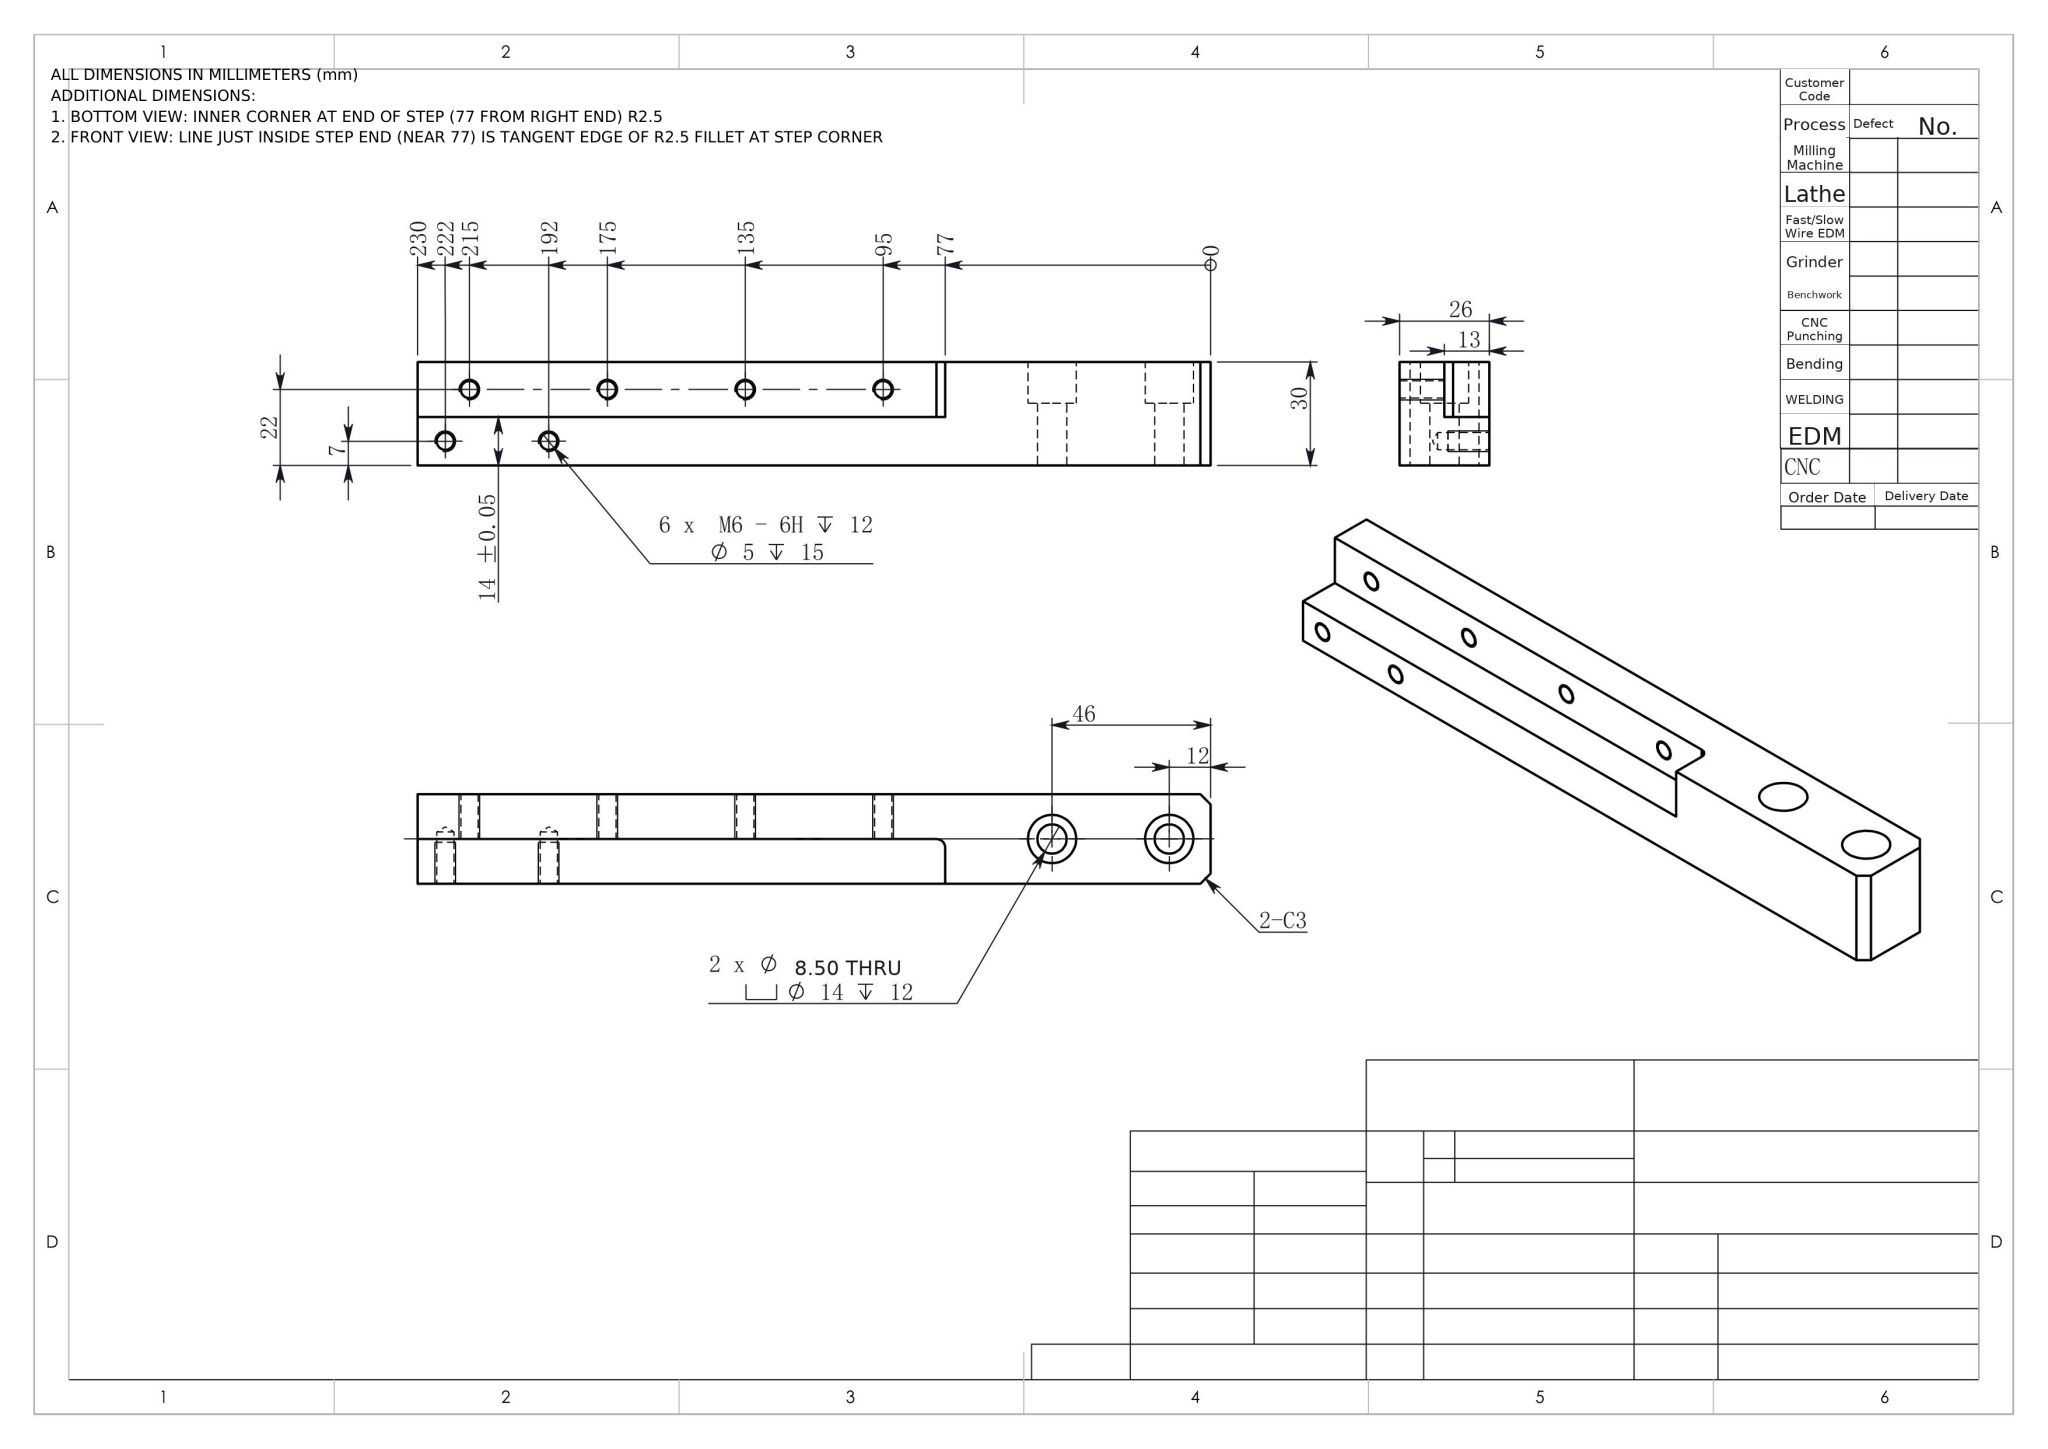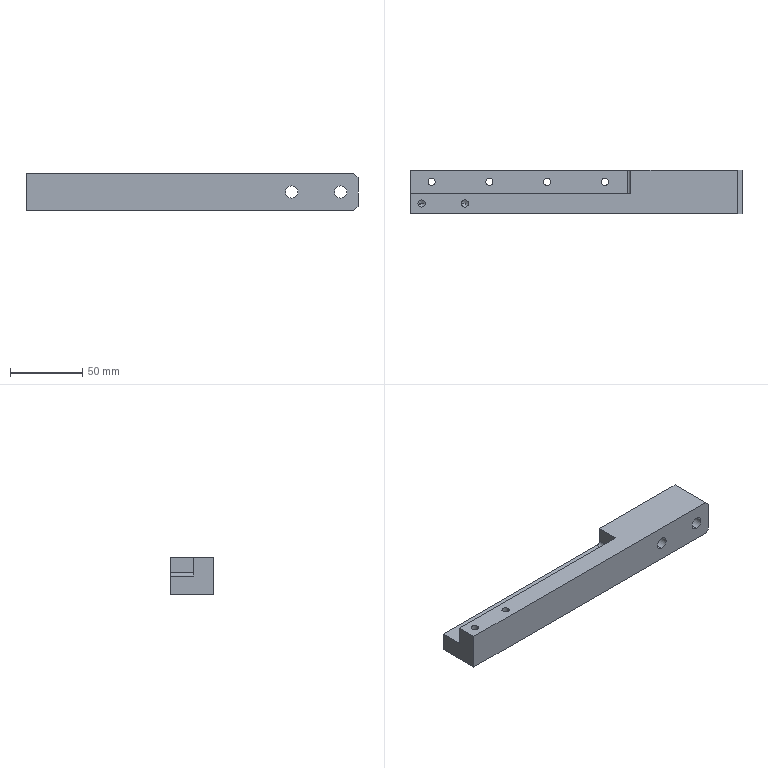Part | NX | mm | 1 solid | 38 faces | box 230 x 30 x 26 mm | volume 139960 mm3 | cylinder 21 | plane 13 | cone 4 | commonest cylinder face diameters 5 x13 14 x4 8.5 x4